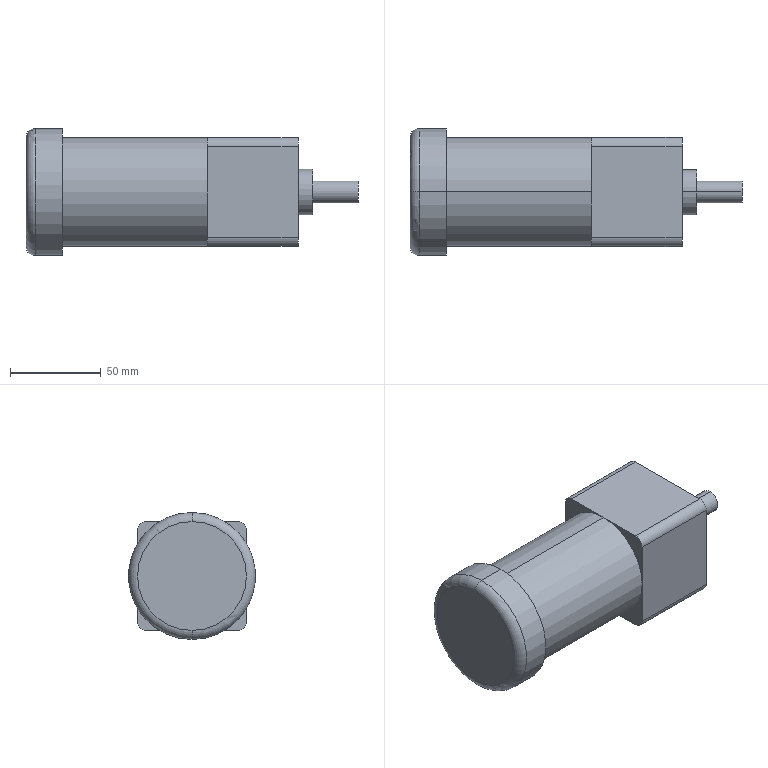Component | SolidWorks | Motor-1 | 1 solid | 27 faces | box 183 x 70 x 70 mm | volume 487703 mm3 | plane 13 | cylinder 12 | torus 2 | commonest cylinder face diameters 10 x4 12 x2 25 x2 70 x2 60 x2 | material Plain Carbon Steel
build123d program:
from build123d import *

# Parameters (mm, degrees)
SKETCH1_W           = 60
SKETCH1_H           = 60
BOSS_EXTRUDE1_DEPTH = 50
SKETCH2_R           = 30
BOSS_EXTRUDE2_DEPTH = 80
SKETCH3_R           = 35
BOSS_EXTRUDE3_DEPTH = 20
SKETCH4_R           = 12.5
BOSS_EXTRUDE4_DEPTH = 8
SKETCH5_R           = 6
BOSS_EXTRUDE5_DEPTH = 25
FILLET1_R           = 5


with BuildPart() as part:
    # Sketch1 → Boss-Extrude1 (new body)
    with BuildSketch(Plane.XY):
        Rectangle(SKETCH1_W, SKETCH1_H)
    extrude(amount=BOSS_EXTRUDE1_DEPTH)

    # Sketch2 → Boss-Extrude2 (add)
    with BuildSketch(Plane(origin=(0, 0, 0), x_dir=(-1, 0, 0), z_dir=(0, 0, -1))):
        Circle(SKETCH2_R)
    extrude(amount=BOSS_EXTRUDE2_DEPTH)

    # Sketch3 → Boss-Extrude3 (add)
    with BuildSketch(Plane(origin=(0, 0, -80), x_dir=(-1, 0, 0), z_dir=(0, 0, -1))):
        Circle(SKETCH3_R)
    extrude(amount=BOSS_EXTRUDE3_DEPTH)

    # Sketch4 → Boss-Extrude4 (add)
    with BuildSketch(Plane.XY.offset(50)):
        Circle(SKETCH4_R)
    extrude(amount=BOSS_EXTRUDE4_DEPTH)

    # Sketch5 → Boss-Extrude5 (add)
    with BuildSketch(Plane.XY.offset(58)):
        Circle(SKETCH5_R)
    extrude(amount=BOSS_EXTRUDE5_DEPTH)

    # Fillet1
    fillet1_edges = [part.edges().sort_by_distance(p)[0] for p in [
        (35, 0, -100),
        (-30, 30, 25),
        (30, 30, 25),
        (30, -30, 25),
        (-30, -30, 25),
    ]]
    fillet(fillet1_edges, radius=FILLET1_R)


solid = part.part

# Placed as in the assembly
solid = solid.moved(Location((-106.55, 5.646, 1535), (0, 90, 0)))
STEP:
#1=COLOUR_RGB('',0.7922,0.8196,0.9333);
#2=FILL_AREA_STYLE_COLOUR('',#1);
#3=FILL_AREA_STYLE('',(#2));
#4=SURFACE_STYLE_FILL_AREA(#3);
#5=SURFACE_SIDE_STYLE('',(#4));
#6=SURFACE_STYLE_USAGE(.BOTH.,#5);
#7=PRESENTATION_STYLE_ASSIGNMENT((#6));
#8=CARTESIAN_POINT('',(-7.935,0.2223,59.055));
#9=VERTEX_POINT('',#8);
#10=CARTESIAN_POINT('',(-7.935,0.2223,61.811));
#11=VERTEX_POINT('',#10);
#12=CARTESIAN_POINT('',(-7.935,0.2223,60.433));
#13=DIRECTION('',(1.,0.,0.));
#14=DIRECTION('',(0.,0.,1.));
#15=AXIS2_PLACEMENT_3D('',#12,#13,#14);
#16=CIRCLE('',#15,1.378);
#17=EDGE_CURVE('',#9,#11,#16,.T.);
#18=ORIENTED_EDGE('',*,*,#17,.F.);
#19=CARTESIAN_POINT('',(-8.132,0.2223,59.252));
#20=VERTEX_POINT('',#19);
#21=CARTESIAN_POINT('',(-7.935,0.2223,59.252));
#22=DIRECTION('',(-0.,1.,0.));
#23=DIRECTION('',(-1.,0.,0.));
#24=AXIS2_PLACEMENT_3D('',#21,#22,#23);
#25=CIRCLE('',#24,0.1969);
#26=EDGE_CURVE('',#9,#20,#25,.T.);
#27=ORIENTED_EDGE('',*,*,#26,.T.);
#28=CARTESIAN_POINT('',(-8.132,0.2223,61.614));
#29=VERTEX_POINT('',#28);
#30=CARTESIAN_POINT('',(-8.132,0.2223,60.433));
#31=DIRECTION('',(-1.,-0.,-0.));
#32=DIRECTION('',(0.,0.,1.));
#33=AXIS2_PLACEMENT_3D('',#30,#31,#32);
#34=CIRCLE('',#33,1.181);
#35=EDGE_CURVE('',#29,#20,#34,.T.);
#36=ORIENTED_EDGE('',*,*,#35,.F.);
#37=CARTESIAN_POINT('',(-7.935,0.2223,61.614));
#38=DIRECTION('',(0.,-1.,0.));
#39=DIRECTION('',(0.,-0.,-1.));
#40=AXIS2_PLACEMENT_3D('',#37,#38,#39);
#41=CIRCLE('',#40,0.1969);
#42=EDGE_CURVE('',#11,#29,#41,.T.);
#43=ORIENTED_EDGE('',*,*,#42,.F.);
#44=EDGE_LOOP('',(#18,#27,#36,#43));
#45=FACE_OUTER_BOUND('',#44,.T.);
#46=CARTESIAN_POINT('',(-7.935,0.2223,60.433));
#47=DIRECTION('',(-1.,-0.,-0.));
#48=DIRECTION('',(-0.,0.,1.));
#49=AXIS2_PLACEMENT_3D('',#46,#47,#48);
#50=TOROIDAL_SURFACE('',#49,1.181,0.1969);
#51=ADVANCED_FACE('',(#45),#50,.T.);
#52=CARTESIAN_POINT('',(-0.9271,0.2223,60.197));
#53=VERTEX_POINT('',#52);
#54=CARTESIAN_POINT('',(-0.9271,0.2223,60.669));
#55=VERTEX_POINT('',#54);
#56=CARTESIAN_POINT('',(-0.9271,0.2223,60.433));
#57=DIRECTION('',(1.,0.,0.));
#58=DIRECTION('',(0.,-0.,-1.));
#59=AXIS2_PLACEMENT_3D('',#56,#57,#58);
#60=CIRCLE('',#59,0.2362);
#61=EDGE_CURVE('',#53,#55,#60,.T.);
#62=ORIENTED_EDGE('',*,*,#61,.F.);
#63=CARTESIAN_POINT('',(-1.911,0.2223,60.197));
#64=VERTEX_POINT('',#63);
#65=CARTESIAN_POINT('',(-0.9271,0.2223,60.197));
#66=DIRECTION('',(-1.,-0.,-0.));
#67=VECTOR('',#66,39.37);
#68=LINE('',#65,#67);
#69=EDGE_CURVE('',#53,#64,#68,.T.);
#70=ORIENTED_EDGE('',*,*,#69,.T.);
#71=CARTESIAN_POINT('',(-1.911,0.2223,60.669));
#72=VERTEX_POINT('',#71);
#73=CARTESIAN_POINT('',(-1.911,0.2223,60.433));
#74=DIRECTION('',(1.,0.,0.));
#75=DIRECTION('',(0.,-0.,-1.));
#76=AXIS2_PLACEMENT_3D('',#73,#74,#75);
#77=CIRCLE('',#76,0.2362);
#78=EDGE_CURVE('',#64,#72,#77,.T.);
#79=ORIENTED_EDGE('',*,*,#78,.T.);
#80=CARTESIAN_POINT('',(-0.9271,0.2223,60.669));
#81=DIRECTION('',(-1.,-0.,-0.));
#82=VECTOR('',#81,39.37);
#83=LINE('',#80,#82);
#84=EDGE_CURVE('',#55,#72,#83,.T.);
#85=ORIENTED_EDGE('',*,*,#84,.F.);
#86=EDGE_LOOP('',(#62,#70,#79,#85));
#87=FACE_OUTER_BOUND('',#86,.T.);
#88=CARTESIAN_POINT('',(-0.9271,0.2223,60.433));
#89=DIRECTION('',(-1.,-0.,-0.));
#90=DIRECTION('',(0.,0.,1.));
#91=AXIS2_PLACEMENT_3D('',#88,#89,#90);
#92=CYLINDRICAL_SURFACE('',#91,0.2362);
#93=ADVANCED_FACE('',(#87),#92,.T.);
#94=CARTESIAN_POINT('',(-1.911,0.2223,59.941));
#95=VERTEX_POINT('',#94);
#96=CARTESIAN_POINT('',(-1.911,0.2223,60.925));
#97=VERTEX_POINT('',#96);
#98=CARTESIAN_POINT('',(-1.911,0.2223,60.433));
#99=DIRECTION('',(1.,0.,0.));
#100=DIRECTION('',(0.,-0.,-1.));
#101=AXIS2_PLACEMENT_3D('',#98,#99,#100);
#102=CIRCLE('',#101,0.4921);
#103=EDGE_CURVE('',#95,#97,#102,.T.);
#104=ORIENTED_EDGE('',*,*,#103,.F.);
#105=CARTESIAN_POINT('',(-2.226,0.2223,59.941));
#106=VERTEX_POINT('',#105);
#107=CARTESIAN_POINT('',(-1.911,0.2223,59.941));
#108=DIRECTION('',(-1.,-0.,-0.));
#109=VECTOR('',#108,39.37);
#110=LINE('',#107,#109);
#111=EDGE_CURVE('',#95,#106,#110,.T.);
#112=ORIENTED_EDGE('',*,*,#111,.T.);
#113=CARTESIAN_POINT('',(-2.226,0.2223,60.925));
#114=VERTEX_POINT('',#113);
#115=CARTESIAN_POINT('',(-2.226,0.2223,60.433));
#116=DIRECTION('',(1.,0.,0.));
#117=DIRECTION('',(0.,-0.,-1.));
#118=AXIS2_PLACEMENT_3D('',#115,#116,#117);
#119=CIRCLE('',#118,0.4921);
#120=EDGE_CURVE('',#106,#114,#119,.T.);
#121=ORIENTED_EDGE('',*,*,#120,.T.);
#122=CARTESIAN_POINT('',(-1.911,0.2223,60.925));
#123=DIRECTION('',(-1.,-0.,-0.));
#124=VECTOR('',#123,39.37);
#125=LINE('',#122,#124);
#126=EDGE_CURVE('',#97,#114,#125,.T.);
#127=ORIENTED_EDGE('',*,*,#126,.F.);
#128=EDGE_LOOP('',(#104,#112,#121,#127));
#129=FACE_OUTER_BOUND('',#128,.T.);
#130=CARTESIAN_POINT('',(-1.911,0.2223,60.433));
#131=DIRECTION('',(-1.,-0.,-0.));
#132=DIRECTION('',(0.,0.,1.));
#133=AXIS2_PLACEMENT_3D('',#130,#131,#132);
#134=CYLINDRICAL_SURFACE('',#133,0.4921);
#135=ADVANCED_FACE('',(#129),#134,.T.);
#136=ORIENTED_EDGE('',*,*,#17,.T.);
#137=CARTESIAN_POINT('',(-7.344,0.2223,61.811));
#138=VERTEX_POINT('',#137);
#139=CARTESIAN_POINT('',(-8.132,0.2223,61.811));
#140=DIRECTION('',(1.,0.,0.));
#141=VECTOR('',#140,39.37);
#142=LINE('',#139,#141);
#143=EDGE_CURVE('',#11,#138,#142,.T.);
#144=ORIENTED_EDGE('',*,*,#143,.T.);
#145=CARTESIAN_POINT('',(-7.344,0.2223,59.055));
#146=VERTEX_POINT('',#145);
#147=CARTESIAN_POINT('',(-7.344,0.2223,60.433));
#148=DIRECTION('',(-1.,-0.,-0.));
#149=DIRECTION('',(0.,0.,1.));
#150=AXIS2_PLACEMENT_3D('',#147,#148,#149);
#151=CIRCLE('',#150,1.378);
#152=EDGE_CURVE('',#138,#146,#151,.T.);
#153=ORIENTED_EDGE('',*,*,#152,.T.);
#154=CARTESIAN_POINT('',(-8.132,0.2223,59.055));
#155=DIRECTION('',(1.,0.,0.));
#156=VECTOR('',#155,39.37);
#157=LINE('',#154,#156);
#158=EDGE_CURVE('',#9,#146,#157,.T.);
#159=ORIENTED_EDGE('',*,*,#158,.F.);
#160=EDGE_LOOP('',(#136,#144,#153,#159));
#161=FACE_OUTER_BOUND('',#160,.T.);
#162=CARTESIAN_POINT('',(-8.132,0.2223,60.433));
#163=DIRECTION('',(1.,0.,0.));
#164=DIRECTION('',(0.,-0.,-1.));
#165=AXIS2_PLACEMENT_3D('',#162,#163,#164);
#166=CYLINDRICAL_SURFACE('',#165,1.378);
#167=ADVANCED_FACE('',(#161),#166,.T.);
#168=CARTESIAN_POINT('',(-7.344,0.2223,61.614));
#169=VERTEX_POINT('',#168);
#170=CARTESIAN_POINT('',(-7.344,0.2223,59.252));
#171=VERTEX_POINT('',#170);
#172=CARTESIAN_POINT('',(-7.344,0.2223,60.433));
#173=DIRECTION('',(-1.,-0.,-0.));
#174=DIRECTION('',(0.,0.,1.));
#175=AXIS2_PLACEMENT_3D('',#172,#173,#174);
#176=CIRCLE('',#175,1.181);
#177=EDGE_CURVE('',#169,#171,#176,.T.);
#178=ORIENTED_EDGE('',*,*,#177,.F.);
#179=CARTESIAN_POINT('',(-4.195,0.2223,61.614));
#180=VERTEX_POINT('',#179);
#181=CARTESIAN_POINT('',(-7.344,0.2223,61.614));
#182=DIRECTION('',(1.,0.,0.));
#183=VECTOR('',#182,39.37);
#184=LINE('',#181,#183);
#185=EDGE_CURVE('',#169,#180,#184,.T.);
#186=ORIENTED_EDGE('',*,*,#185,.T.);
#187=CARTESIAN_POINT('',(-4.195,1.403,60.433));
#188=VERTEX_POINT('',#187);
#189=CARTESIAN_POINT('',(-4.195,0.2223,60.433));
#190=DIRECTION('',(-1.,-0.,-0.));
#191=DIRECTION('',(0.,0.,1.));
#192=AXIS2_PLACEMENT_3D('',#189,#190,#191);
#193=CIRCLE('',#192,1.181);
#194=EDGE_CURVE('',#180,#188,#193,.T.);
#195=ORIENTED_EDGE('',*,*,#194,.T.);
#196=CARTESIAN_POINT('',(-4.195,0.2223,59.252));
#197=VERTEX_POINT('',#196);
#198=CARTESIAN_POINT('',(-4.195,0.2223,60.433));
#199=DIRECTION('',(-1.,-0.,-0.));
#200=DIRECTION('',(0.,0.,1.));
#201=AXIS2_PLACEMENT_3D('',#198,#199,#200);
#202=CIRCLE('',#201,1.181);
#203=EDGE_CURVE('',#188,#197,#202,.T.);
#204=ORIENTED_EDGE('',*,*,#203,.T.);
#205=CARTESIAN_POINT('',(-7.344,0.2223,59.252));
#206=DIRECTION('',(1.,0.,0.));
#207=VECTOR('',#206,39.37);
#208=LINE('',#205,#207);
#209=EDGE_CURVE('',#171,#197,#208,.T.);
#210=ORIENTED_EDGE('',*,*,#209,.F.);
#211=EDGE_LOOP('',(#178,#186,#195,#204,#210));
#212=FACE_OUTER_BOUND('',#211,.T.);
#213=CARTESIAN_POINT('',(-7.344,0.2223,60.433));
#214=DIRECTION('',(1.,0.,0.));
#215=DIRECTION('',(0.,-0.,-1.));
#216=AXIS2_PLACEMENT_3D('',#213,#214,#215);
#217=CYLINDRICAL_SURFACE('',#216,1.181);
#218=ADVANCED_FACE('',(#212),#217,.T.);
#219=CARTESIAN_POINT('',(-1.911,0.2223,60.433));
#220=DIRECTION('',(1.,0.,0.));
#221=DIRECTION('',(0.,-0.,-1.));
#222=AXIS2_PLACEMENT_3D('',#219,#220,#221);
#223=CIRCLE('',#222,0.4921);
#224=EDGE_CURVE('',#97,#95,#223,.T.);
#225=ORIENTED_EDGE('',*,*,#224,.T.);
#226=ORIENTED_EDGE('',*,*,#103,.T.);
#227=EDGE_LOOP('',(#225,#226));
#228=FACE_OUTER_BOUND('',#227,.T.);
#229=CARTESIAN_POINT('',(-1.911,0.2223,60.433));
#230=DIRECTION('',(1.,0.,0.));
#231=DIRECTION('',(0.,-0.,-1.));
#232=AXIS2_PLACEMENT_3D('',#229,#230,#231);
#233=CIRCLE('',#232,0.2362);
#234=EDGE_CURVE('',#72,#64,#233,.T.);
#235=ORIENTED_EDGE('',*,*,#234,.F.);
#236=ORIENTED_EDGE('',*,*,#78,.F.);
#237=EDGE_LOOP('',(#235,#236));
#238=FACE_BOUND('',#237,.T.);
#239=CARTESIAN_POINT('',(-1.911,0.2223,60.433));
#240=DIRECTION('',(1.,0.,0.));
#241=DIRECTION('',(0.,-0.,-1.));
#242=AXIS2_PLACEMENT_3D('',#239,#240,#241);
#243=PLANE('',#242);
#244=ADVANCED_FACE('',(#228,#238),#243,.T.);
#245=CARTESIAN_POINT('',(-2.226,-0.9588,61.417));
#246=VERTEX_POINT('',#245);
#247=CARTESIAN_POINT('',(-2.226,-0.9588,59.449));
#248=VERTEX_POINT('',#247);
#249=CARTESIAN_POINT('',(-2.226,-0.9588,59.252));
#250=DIRECTION('',(0.,-0.,-1.));
#251=VECTOR('',#250,39.37);
#252=LINE('',#249,#251);
#253=EDGE_CURVE('',#246,#248,#252,.T.);
#254=ORIENTED_EDGE('',*,*,#253,.T.);
#255=CARTESIAN_POINT('',(-2.226,-0.762,59.252));
#256=VERTEX_POINT('',#255);
#257=CARTESIAN_POINT('',(-2.226,-0.762,59.449));
#258=DIRECTION('',(1.,0.,0.));
#259=DIRECTION('',(0.,0.,-1.));
#260=AXIS2_PLACEMENT_3D('',#257,#258,#259);
#261=CIRCLE('',#260,0.1969);
#262=EDGE_CURVE('',#248,#256,#261,.T.);
#263=ORIENTED_EDGE('',*,*,#262,.T.);
#264=CARTESIAN_POINT('',(-2.226,1.207,59.252));
#265=VERTEX_POINT('',#264);
#266=CARTESIAN_POINT('',(-2.226,-0.9588,59.252));
#267=DIRECTION('',(-0.,1.,-0.));
#268=VECTOR('',#267,39.37);
#269=LINE('',#266,#268);
#270=EDGE_CURVE('',#256,#265,#269,.T.);
#271=ORIENTED_EDGE('',*,*,#270,.T.);
#272=CARTESIAN_POINT('',(-2.226,1.403,59.449));
#273=VERTEX_POINT('',#272);
#274=CARTESIAN_POINT('',(-2.226,1.207,59.449));
#275=DIRECTION('',(1.,0.,0.));
#276=DIRECTION('',(0.,0.,-1.));
#277=AXIS2_PLACEMENT_3D('',#274,#275,#276);
#278=CIRCLE('',#277,0.1969);
#279=EDGE_CURVE('',#265,#273,#278,.T.);
#280=ORIENTED_EDGE('',*,*,#279,.T.);
#281=CARTESIAN_POINT('',(-2.226,1.403,61.417));
#282=VERTEX_POINT('',#281);
#283=CARTESIAN_POINT('',(-2.226,1.403,59.252));
#284=DIRECTION('',(-0.,0.,1.));
#285=VECTOR('',#284,39.37);
#286=LINE('',#283,#285);
#287=EDGE_CURVE('',#273,#282,#286,.T.);
#288=ORIENTED_EDGE('',*,*,#287,.T.);
#289=CARTESIAN_POINT('',(-2.226,1.207,61.614));
#290=VERTEX_POINT('',#289);
#291=CARTESIAN_POINT('',(-2.226,1.207,61.417));
#292=DIRECTION('',(1.,0.,0.));
#293=DIRECTION('',(0.,0.,-1.));
#294=AXIS2_PLACEMENT_3D('',#291,#292,#293);
#295=CIRCLE('',#294,0.1969);
#296=EDGE_CURVE('',#282,#290,#295,.T.);
#297=ORIENTED_EDGE('',*,*,#296,.T.);
#298=CARTESIAN_POINT('',(-2.226,-0.762,61.614));
#299=VERTEX_POINT('',#298);
#300=CARTESIAN_POINT('',(-2.226,-0.9588,61.614));
#301=DIRECTION('',(0.,-1.,0.));
#302=VECTOR('',#301,39.37);
#303=LINE('',#300,#302);
#304=EDGE_CURVE('',#290,#299,#303,.T.);
#305=ORIENTED_EDGE('',*,*,#304,.T.);
#306=CARTESIAN_POINT('',(-2.226,-0.762,61.417));
#307=DIRECTION('',(1.,0.,0.));
#308=DIRECTION('',(0.,0.,-1.));
#309=AXIS2_PLACEMENT_3D('',#306,#307,#308);
#310=CIRCLE('',#309,0.1969);
#311=EDGE_CURVE('',#299,#246,#310,.T.);
#312=ORIENTED_EDGE('',*,*,#311,.T.);
#313=EDGE_LOOP('',(#254,#263,#271,#280,#288,#297,#305,#312));
#314=FACE_OUTER_BOUND('',#313,.T.);
#315=CARTESIAN_POINT('',(-2.226,0.2223,60.433));
#316=DIRECTION('',(1.,0.,0.));
#317=DIRECTION('',(0.,-0.,-1.));
#318=AXIS2_PLACEMENT_3D('',#315,#316,#317);
#319=CIRCLE('',#318,0.4921);
#320=EDGE_CURVE('',#114,#106,#319,.T.);
#321=ORIENTED_EDGE('',*,*,#320,.F.);
#322=ORIENTED_EDGE('',*,*,#120,.F.);
#323=EDGE_LOOP('',(#321,#322));
#324=FACE_BOUND('',#323,.T.);
#325=CARTESIAN_POINT('',(-2.226,0.2223,60.433));
#326=DIRECTION('',(1.,0.,0.));
#327=DIRECTION('',(0.,-0.,-1.));
#328=AXIS2_PLACEMENT_3D('',#325,#326,#327);
#329=PLANE('',#328);
#330=ADVANCED_FACE('',(#314,#324),#329,.T.);
#331=CARTESIAN_POINT('',(-4.195,1.207,61.614));
#332=VERTEX_POINT('',#331);
#333=CARTESIAN_POINT('',(-4.195,-0.9588,61.614));
#334=DIRECTION('',(0.,-1.,0.));
#335=VECTOR('',#334,39.37);
#336=LINE('',#333,#335);
#337=EDGE_CURVE('',#332,#180,#336,.T.);
#338=ORIENTED_EDGE('',*,*,#337,.F.);
#339=CARTESIAN_POINT('',(-4.195,1.403,61.417));
#340=VERTEX_POINT('',#339);
#341=CARTESIAN_POINT('',(-4.195,1.207,61.417));
#342=DIRECTION('',(-1.,-0.,-0.));
#343=DIRECTION('',(0.,0.,-1.));
#344=AXIS2_PLACEMENT_3D('',#341,#342,#343);
#345=CIRCLE('',#344,0.1969);
#346=EDGE_CURVE('',#332,#340,#345,.T.);
#347=ORIENTED_EDGE('',*,*,#346,.T.);
#348=CARTESIAN_POINT('',(-4.195,1.403,59.252));
#349=DIRECTION('',(-0.,0.,1.));
#350=VECTOR('',#349,39.37);
#351=LINE('',#348,#350);
#352=EDGE_CURVE('',#188,#340,#351,.T.);
#353=ORIENTED_EDGE('',*,*,#352,.F.);
#354=ORIENTED_EDGE('',*,*,#194,.F.);
#355=EDGE_LOOP('',(#338,#347,#353,#354));
#356=FACE_OUTER_BOUND('',#355,.T.);
#357=CARTESIAN_POINT('',(-4.195,0.2223,60.433));
#358=DIRECTION('',(1.,0.,0.));
#359=DIRECTION('',(0.,-0.,-1.));
#360=AXIS2_PLACEMENT_3D('',#357,#358,#359);
#361=PLANE('',#360);
#362=ADVANCED_FACE('',(#356),#361,.F.);
#363=CARTESIAN_POINT('',(-4.195,1.403,59.449));
#364=VERTEX_POINT('',#363);
#365=CARTESIAN_POINT('',(-4.195,1.403,59.252));
#366=DIRECTION('',(-0.,0.,1.));
#367=VECTOR('',#366,39.37);
#368=LINE('',#365,#367);
#369=EDGE_CURVE('',#364,#188,#368,.T.);
#370=ORIENTED_EDGE('',*,*,#369,.F.);
#371=CARTESIAN_POINT('',(-4.195,1.207,59.252));
#372=VERTEX_POINT('',#371);
#373=CARTESIAN_POINT('',(-4.195,1.207,59.449));
#374=DIRECTION('',(-1.,-0.,-0.));
#375=DIRECTION('',(0.,0.,-1.));
#376=AXIS2_PLACEMENT_3D('',#373,#374,#375);
#377=CIRCLE('',#376,0.1969);
#378=EDGE_CURVE('',#364,#372,#377,.T.);
#379=ORIENTED_EDGE('',*,*,#378,.T.);
#380=CARTESIAN_POINT('',(-4.195,-0.9588,59.252));
#381=DIRECTION('',(-0.,1.,-0.));
#382=VECTOR('',#381,39.37);
#383=LINE('',#380,#382);
#384=EDGE_CURVE('',#197,#372,#383,.T.);
#385=ORIENTED_EDGE('',*,*,#384,.F.);
#386=ORIENTED_EDGE('',*,*,#203,.F.);
#387=EDGE_LOOP('',(#370,#379,#385,#386));
#388=FACE_OUTER_BOUND('',#387,.T.);
#389=CARTESIAN_POINT('',(-4.195,0.2223,60.433));
#390=DIRECTION('',(1.,0.,0.));
#391=DIRECTION('',(0.,-0.,-1.));
#392=AXIS2_PLACEMENT_3D('',#389,#390,#391);
#393=PLANE('',#392);
#394=ADVANCED_FACE('',(#388),#393,.F.);
#395=CARTESIAN_POINT('',(-4.195,-0.762,59.252));
#396=VERTEX_POINT('',#395);
#397=CARTESIAN_POINT('',(-4.195,-0.9588,59.252));
#398=DIRECTION('',(-0.,1.,-0.));
#399=VECTOR('',#398,39.37);
#400=LINE('',#397,#399);
#401=EDGE_CURVE('',#396,#197,#400,.T.);
#402=ORIENTED_EDGE('',*,*,#401,.F.);
#403=CARTESIAN_POINT('',(-4.195,-0.9588,59.449));
#404=VERTEX_POINT('',#403);
#405=CARTESIAN_POINT('',(-4.195,-0.762,59.449));
#406=DIRECTION('',(-1.,-0.,-0.));
#407=DIRECTION('',(0.,0.,-1.));
#408=AXIS2_PLACEMENT_3D('',#405,#406,#407);
#409=CIRCLE('',#408,0.1969);
#410=EDGE_CURVE('',#396,#404,#409,.T.);
#411=ORIENTED_EDGE('',*,*,#410,.T.);
#412=CARTESIAN_POINT('',(-4.195,-0.9588,60.433));
#413=VERTEX_POINT('',#412);
#414=CARTESIAN_POINT('',(-4.195,-0.9588,59.252));
#415=DIRECTION('',(0.,-0.,-1.));
#416=VECTOR('',#415,39.37);
#417=LINE('',#414,#416);
#418=EDGE_CURVE('',#413,#404,#417,.T.);
#419=ORIENTED_EDGE('',*,*,#418,.F.);
#420=CARTESIAN_POINT('',(-4.195,0.2223,60.433));
#421=DIRECTION('',(-1.,-0.,-0.));
#422=DIRECTION('',(0.,0.,1.));
#423=AXIS2_PLACEMENT_3D('',#420,#421,#422);
#424=CIRCLE('',#423,1.181);
#425=EDGE_CURVE('',#197,#413,#424,.T.);
#426=ORIENTED_EDGE('',*,*,#425,.F.);
#427=EDGE_LOOP('',(#402,#411,#419,#426));
#428=FACE_OUTER_BOUND('',#427,.T.);
#429=CARTESIAN_POINT('',(-4.195,0.2223,60.433));
#430=DIRECTION('',(1.,0.,0.));
#431=DIRECTION('',(0.,-0.,-1.));
#432=AXIS2_PLACEMENT_3D('',#429,#430,#431);
#433=PLANE('',#432);
#434=ADVANCED_FACE('',(#428),#433,.F.);
#435=CARTESIAN_POINT('',(-4.195,-0.9588,61.417));
#436=VERTEX_POINT('',#435);
#437=CARTESIAN_POINT('',(-4.195,-0.9588,59.252));
#438=DIRECTION('',(0.,-0.,-1.));
#439=VECTOR('',#438,39.37);
#440=LINE('',#437,#439);
#441=EDGE_CURVE('',#436,#413,#440,.T.);
#442=ORIENTED_EDGE('',*,*,#441,.F.);
#443=CARTESIAN_POINT('',(-4.195,-0.762,61.614));
#444=VERTEX_POINT('',#443);
#445=CARTESIAN_POINT('',(-4.195,-0.762,61.417));
#446=DIRECTION('',(-1.,-0.,-0.));
#447=DIRECTION('',(0.,0.,-1.));
#448=AXIS2_PLACEMENT_3D('',#445,#446,#447);
#449=CIRCLE('',#448,0.1969);
#450=EDGE_CURVE('',#436,#444,#449,.T.);
#451=ORIENTED_EDGE('',*,*,#450,.T.);
#452=CARTESIAN_POINT('',(-4.195,-0.9588,61.614));
#453=DIRECTION('',(0.,-1.,0.));
#454=VECTOR('',#453,39.37);
#455=LINE('',#452,#454);
#456=EDGE_CURVE('',#180,#444,#455,.T.);
#457=ORIENTED_EDGE('',*,*,#456,.F.);
#458=CARTESIAN_POINT('',(-4.195,0.2223,60.433));
#459=DIRECTION('',(-1.,-0.,-0.));
#460=DIRECTION('',(0.,0.,1.));
#461=AXIS2_PLACEMENT_3D('',#458,#459,#460);
#462=CIRCLE('',#461,1.181);
#463=EDGE_CURVE('',#413,#180,#462,.T.);
#464=ORIENTED_EDGE('',*,*,#463,.F.);
#465=EDGE_LOOP('',(#442,#451,#457,#464));
#466=FACE_OUTER_BOUND('',#465,.T.);
#467=CARTESIAN_POINT('',(-4.195,0.2223,60.433));
#468=DIRECTION('',(1.,0.,0.));
#469=DIRECTION('',(0.,-0.,-1.));
#470=AXIS2_PLACEMENT_3D('',#467,#468,#469);
#471=PLANE('',#470);
#472=ADVANCED_FACE('',(#466),#471,.F.);
#473=ORIENTED_EDGE('',*,*,#456,.T.);
#474=CARTESIAN_POINT('',(-2.226,-0.762,61.614));
#475=DIRECTION('',(1.,0.,0.));
#476=VECTOR('',#475,39.37);
#477=LINE('',#474,#476);
#478=EDGE_CURVE('',#444,#299,#477,.T.);
#479=ORIENTED_EDGE('',*,*,#478,.T.);
#480=ORIENTED_EDGE('',*,*,#304,.F.);
#481=CARTESIAN_POINT('',(-2.226,1.207,61.614));
#482=DIRECTION('',(-1.,-0.,-0.));
#483=VECTOR('',#482,39.37);
#484=LINE('',#481,#483);
#485=EDGE_CURVE('',#290,#332,#484,.T.);
#486=ORIENTED_EDGE('',*,*,#485,.T.);
#487=ORIENTED_EDGE('',*,*,#337,.T.);
#488=EDGE_LOOP('',(#473,#479,#480,#486,#487));
#489=FACE_OUTER_BOUND('',#488,.T.);
#490=CARTESIAN_POINT('',(-2.226,-0.9588,61.614));
#491=DIRECTION('',(0.,-0.,-1.));
#492=DIRECTION('',(-1.,-0.,-0.));
#493=AXIS2_PLACEMENT_3D('',#490,#491,#492);
#494=PLANE('',#493);
#495=ADVANCED_FACE('',(#489),#494,.F.);
#496=ORIENTED_EDGE('',*,*,#418,.T.);
#497=CARTESIAN_POINT('',(-2.226,-0.9588,59.449));
#498=DIRECTION('',(1.,0.,0.));
#499=VECTOR('',#498,39.37);
#500=LINE('',#497,#499);
#501=EDGE_CURVE('',#404,#248,#500,.T.);
#502=ORIENTED_EDGE('',*,*,#501,.T.);
#503=ORIENTED_EDGE('',*,*,#253,.F.);
#504=CARTESIAN_POINT('',(-2.226,-0.9588,61.417));
#505=DIRECTION('',(-1.,-0.,-0.));
#506=VECTOR('',#505,39.37);
#507=LINE('',#504,#506);
#508=EDGE_CURVE('',#246,#436,#507,.T.);
#509=ORIENTED_EDGE('',*,*,#508,.T.);
#510=ORIENTED_EDGE('',*,*,#441,.T.);
#511=EDGE_LOOP('',(#496,#502,#503,#509,#510));
#512=FACE_OUTER_BOUND('',#511,.T.);
#513=CARTESIAN_POINT('',(-2.226,-0.9588,59.252));
#514=DIRECTION('',(-0.,1.,-0.));
#515=DIRECTION('',(1.,0.,0.));
#516=AXIS2_PLACEMENT_3D('',#513,#514,#515);
#517=PLANE('',#516);
#518=ADVANCED_FACE('',(#512),#517,.F.);
#519=ORIENTED_EDGE('',*,*,#270,.F.);
#520=CARTESIAN_POINT('',(-2.226,-0.762,59.252));
#521=DIRECTION('',(-1.,-0.,-0.));
#522=VECTOR('',#521,39.37);
#523=LINE('',#520,#522);
#524=EDGE_CURVE('',#256,#396,#523,.T.);
#525=ORIENTED_EDGE('',*,*,#524,.T.);
#526=ORIENTED_EDGE('',*,*,#401,.T.);
#527=ORIENTED_EDGE('',*,*,#384,.T.);
#528=CARTESIAN_POINT('',(-2.226,1.207,59.252));
#529=DIRECTION('',(1.,0.,0.));
#530=VECTOR('',#529,39.37);
#531=LINE('',#528,#530);
#532=EDGE_CURVE('',#372,#265,#531,.T.);
#533=ORIENTED_EDGE('',*,*,#532,.T.);
#534=EDGE_LOOP('',(#519,#525,#526,#527,#533));
#535=FACE_OUTER_BOUND('',#534,.T.);
#536=CARTESIAN_POINT('',(-2.226,-0.9588,59.252));
#537=DIRECTION('',(-0.,0.,1.));
#538=DIRECTION('',(1.,0.,0.));
#539=AXIS2_PLACEMENT_3D('',#536,#537,#538);
#540=PLANE('',#539);
#541=ADVANCED_FACE('',(#535),#540,.F.);
#542=ORIENTED_EDGE('',*,*,#352,.T.);
#543=CARTESIAN_POINT('',(-2.226,1.403,61.417));
#544=DIRECTION('',(1.,0.,0.));
#545=VECTOR('',#544,39.37);
#546=LINE('',#543,#545);
#547=EDGE_CURVE('',#340,#282,#546,.T.);
#548=ORIENTED_EDGE('',*,*,#547,.T.);
#549=ORIENTED_EDGE('',*,*,#287,.F.);
#550=CARTESIAN_POINT('',(-2.226,1.403,59.449));
#551=DIRECTION('',(-1.,-0.,-0.));
#552=VECTOR('',#551,39.37);
#553=LINE('',#550,#552);
#554=EDGE_CURVE('',#273,#364,#553,.T.);
#555=ORIENTED_EDGE('',*,*,#554,.T.);
#556=ORIENTED_EDGE('',*,*,#369,.T.);
#557=EDGE_LOOP('',(#542,#548,#549,#555,#556));
#558=FACE_OUTER_BOUND('',#557,.T.);
#559=CARTESIAN_POINT('',(-2.226,1.403,59.252));
#560=DIRECTION('',(0.,-1.,0.));
#561=DIRECTION('',(-1.,-0.,-0.));
#562=AXIS2_PLACEMENT_3D('',#559,#560,#561);
#563=PLANE('',#562);
#564=ADVANCED_FACE('',(#558),#563,.F.);
#565=ORIENTED_EDGE('',*,*,#185,.F.);
#566=CARTESIAN_POINT('',(-7.344,0.2223,60.433));
#567=DIRECTION('',(-1.,-0.,-0.));
#568=DIRECTION('',(0.,0.,1.));
#569=AXIS2_PLACEMENT_3D('',#566,#567,#568);
#570=CIRCLE('',#569,1.181);
#571=EDGE_CURVE('',#171,#169,#570,.T.);
#572=ORIENTED_EDGE('',*,*,#571,.F.);
#573=ORIENTED_EDGE('',*,*,#209,.T.);
#574=ORIENTED_EDGE('',*,*,#425,.T.);
#575=ORIENTED_EDGE('',*,*,#463,.T.);
#576=EDGE_LOOP('',(#565,#572,#573,#574,#575));
#577=FACE_OUTER_BOUND('',#576,.T.);
#578=CARTESIAN_POINT('',(-7.344,0.2223,60.433));
#579=DIRECTION('',(1.,0.,0.));
#580=DIRECTION('',(0.,-0.,-1.));
#581=AXIS2_PLACEMENT_3D('',#578,#579,#580);
#582=CYLINDRICAL_SURFACE('',#581,1.181);
#583=ADVANCED_FACE('',(#577),#582,.T.);
#584=CARTESIAN_POINT('',(-7.344,0.2223,60.433));
#585=DIRECTION('',(-1.,-0.,-0.));
#586=DIRECTION('',(0.,0.,1.));
#587=AXIS2_PLACEMENT_3D('',#584,#585,#586);
#588=CIRCLE('',#587,1.378);
#589=EDGE_CURVE('',#146,#138,#588,.T.);
#590=ORIENTED_EDGE('',*,*,#589,.F.);
#591=ORIENTED_EDGE('',*,*,#152,.F.);
#592=EDGE_LOOP('',(#590,#591));
#593=FACE_OUTER_BOUND('',#592,.T.);
#594=ORIENTED_EDGE('',*,*,#571,.T.);
#595=ORIENTED_EDGE('',*,*,#177,.T.);
#596=EDGE_LOOP('',(#594,#595));
#597=FACE_BOUND('',#596,.T.);
#598=CARTESIAN_POINT('',(-7.344,0.2223,60.433));
#599=DIRECTION('',(-1.,-0.,-0.));
#600=DIRECTION('',(-0.,0.,1.));
#601=AXIS2_PLACEMENT_3D('',#598,#599,#600);
#602=PLANE('',#601);
#603=ADVANCED_FACE('',(#593,#597),#602,.F.);
#604=ORIENTED_EDGE('',*,*,#143,.F.);
#605=CARTESIAN_POINT('',(-7.935,0.2223,60.433));
#606=DIRECTION('',(1.,0.,0.));
#607=DIRECTION('',(0.,0.,1.));
#608=AXIS2_PLACEMENT_3D('',#605,#606,#607);
#609=CIRCLE('',#608,1.378);
#610=EDGE_CURVE('',#11,#9,#609,.T.);
#611=ORIENTED_EDGE('',*,*,#610,.T.);
#612=ORIENTED_EDGE('',*,*,#158,.T.);
#613=ORIENTED_EDGE('',*,*,#589,.T.);
#614=EDGE_LOOP('',(#604,#611,#612,#613));
#615=FACE_OUTER_BOUND('',#614,.T.);
#616=CARTESIAN_POINT('',(-8.132,0.2223,60.433));
#617=DIRECTION('',(1.,0.,0.));
#618=DIRECTION('',(0.,-0.,-1.));
#619=AXIS2_PLACEMENT_3D('',#616,#617,#618);
#620=CYLINDRICAL_SURFACE('',#619,1.378);
#621=ADVANCED_FACE('',(#615),#620,.T.);
#622=ORIENTED_EDGE('',*,*,#35,.T.);
#623=CARTESIAN_POINT('',(-8.132,0.2223,60.433));
#624=DIRECTION('',(-1.,-0.,-0.));
#625=DIRECTION('',(0.,0.,1.));
#626=AXIS2_PLACEMENT_3D('',#623,#624,#625);
#627=CIRCLE('',#626,1.181);
#628=EDGE_CURVE('',#20,#29,#627,.T.);
#629=ORIENTED_EDGE('',*,*,#628,.T.);
#630=EDGE_LOOP('',(#622,#629));
#631=FACE_OUTER_BOUND('',#630,.T.);
#632=CARTESIAN_POINT('',(-8.132,0.2223,60.433));
#633=DIRECTION('',(-1.,-0.,-0.));
#634=DIRECTION('',(-0.,0.,1.));
#635=AXIS2_PLACEMENT_3D('',#632,#633,#634);
#636=PLANE('',#635);
#637=ADVANCED_FACE('',(#631),#636,.T.);
#638=ORIENTED_EDGE('',*,*,#111,.F.);
#639=ORIENTED_EDGE('',*,*,#224,.F.);
#640=ORIENTED_EDGE('',*,*,#126,.T.);
#641=ORIENTED_EDGE('',*,*,#320,.T.);
#642=EDGE_LOOP('',(#638,#639,#640,#641));
#643=FACE_OUTER_BOUND('',#642,.T.);
#644=CARTESIAN_POINT('',(-1.911,0.2223,60.433));
#645=DIRECTION('',(-1.,-0.,-0.));
#646=DIRECTION('',(0.,0.,1.));
#647=AXIS2_PLACEMENT_3D('',#644,#645,#646);
#648=CYLINDRICAL_SURFACE('',#647,0.4921);
#649=ADVANCED_FACE('',(#643),#648,.T.);
#650=ORIENTED_EDGE('',*,*,#69,.F.);
#651=CARTESIAN_POINT('',(-0.9271,0.2223,60.433));
#652=DIRECTION('',(1.,0.,0.));
#653=DIRECTION('',(0.,-0.,-1.));
#654=AXIS2_PLACEMENT_3D('',#651,#652,#653);
#655=CIRCLE('',#654,0.2362);
#656=EDGE_CURVE('',#55,#53,#655,.T.);
#657=ORIENTED_EDGE('',*,*,#656,.F.);
#658=ORIENTED_EDGE('',*,*,#84,.T.);
#659=ORIENTED_EDGE('',*,*,#234,.T.);
#660=EDGE_LOOP('',(#650,#657,#658,#659));
#661=FACE_OUTER_BOUND('',#660,.T.);
#662=CARTESIAN_POINT('',(-0.9271,0.2223,60.433));
#663=DIRECTION('',(-1.,-0.,-0.));
#664=DIRECTION('',(0.,0.,1.));
#665=AXIS2_PLACEMENT_3D('',#662,#663,#664);
#666=CYLINDRICAL_SURFACE('',#665,0.2362);
#667=ADVANCED_FACE('',(#661),#666,.T.);
#668=ORIENTED_EDGE('',*,*,#656,.T.);
#669=ORIENTED_EDGE('',*,*,#61,.T.);
#670=EDGE_LOOP('',(#668,#669));
#671=FACE_OUTER_BOUND('',#670,.T.);
#672=CARTESIAN_POINT('',(-0.9271,0.2223,60.433));
#673=DIRECTION('',(1.,0.,0.));
#674=DIRECTION('',(0.,-0.,-1.));
#675=AXIS2_PLACEMENT_3D('',#672,#673,#674);
#676=PLANE('',#675);
#677=ADVANCED_FACE('',(#671),#676,.T.);
#678=ORIENTED_EDGE('',*,*,#26,.F.);
#679=ORIENTED_EDGE('',*,*,#610,.F.);
#680=ORIENTED_EDGE('',*,*,#42,.T.);
#681=ORIENTED_EDGE('',*,*,#628,.F.);
#682=EDGE_LOOP('',(#678,#679,#680,#681));
#683=FACE_OUTER_BOUND('',#682,.T.);
#684=CARTESIAN_POINT('',(-7.935,0.2223,60.433));
#685=DIRECTION('',(-1.,-0.,-0.));
#686=DIRECTION('',(-0.,0.,1.));
#687=AXIS2_PLACEMENT_3D('',#684,#685,#686);
#688=TOROIDAL_SURFACE('',#687,1.181,0.1969);
#689=ADVANCED_FACE('',(#683),#688,.T.);
#690=ORIENTED_EDGE('',*,*,#262,.F.);
#691=ORIENTED_EDGE('',*,*,#501,.F.);
#692=ORIENTED_EDGE('',*,*,#410,.F.);
#693=ORIENTED_EDGE('',*,*,#524,.F.);
#694=EDGE_LOOP('',(#690,#691,#692,#693));
#695=FACE_OUTER_BOUND('',#694,.T.);
#696=CARTESIAN_POINT('',(-2.226,-0.762,59.449));
#697=DIRECTION('',(-1.,-0.,-0.));
#698=DIRECTION('',(0.,0.,1.));
#699=AXIS2_PLACEMENT_3D('',#696,#697,#698);
#700=CYLINDRICAL_SURFACE('',#699,0.1969);
#701=ADVANCED_FACE('',(#695),#700,.T.);
#702=ORIENTED_EDGE('',*,*,#311,.F.);
#703=ORIENTED_EDGE('',*,*,#478,.F.);
#704=ORIENTED_EDGE('',*,*,#450,.F.);
#705=ORIENTED_EDGE('',*,*,#508,.F.);
#706=EDGE_LOOP('',(#702,#703,#704,#705));
#707=FACE_OUTER_BOUND('',#706,.T.);
#708=CARTESIAN_POINT('',(-2.226,-0.762,61.417));
#709=DIRECTION('',(-1.,-0.,-0.));
#710=DIRECTION('',(0.,0.,1.));
#711=AXIS2_PLACEMENT_3D('',#708,#709,#710);
#712=CYLINDRICAL_SURFACE('',#711,0.1969);
#713=ADVANCED_FACE('',(#707),#712,.T.);
#714=ORIENTED_EDGE('',*,*,#296,.F.);
#715=ORIENTED_EDGE('',*,*,#547,.F.);
#716=ORIENTED_EDGE('',*,*,#346,.F.);
#717=ORIENTED_EDGE('',*,*,#485,.F.);
#718=EDGE_LOOP('',(#714,#715,#716,#717));
#719=FACE_OUTER_BOUND('',#718,.T.);
#720=CARTESIAN_POINT('',(-2.226,1.207,61.417));
#721=DIRECTION('',(-1.,-0.,-0.));
#722=DIRECTION('',(0.,0.,1.));
#723=AXIS2_PLACEMENT_3D('',#720,#721,#722);
#724=CYLINDRICAL_SURFACE('',#723,0.1969);
#725=ADVANCED_FACE('',(#719),#724,.T.);
#726=ORIENTED_EDGE('',*,*,#279,.F.);
#727=ORIENTED_EDGE('',*,*,#532,.F.);
#728=ORIENTED_EDGE('',*,*,#378,.F.);
#729=ORIENTED_EDGE('',*,*,#554,.F.);
#730=EDGE_LOOP('',(#726,#727,#728,#729));
#731=FACE_OUTER_BOUND('',#730,.T.);
#732=CARTESIAN_POINT('',(-2.226,1.207,59.449));
#733=DIRECTION('',(-1.,-0.,-0.));
#734=DIRECTION('',(0.,0.,1.));
#735=AXIS2_PLACEMENT_3D('',#732,#733,#734);
#736=CYLINDRICAL_SURFACE('',#735,0.1969);
#737=ADVANCED_FACE('',(#731),#736,.T.);
#738=CLOSED_SHELL('',(#51,#93,#135,#167,#218,#244,#330,#362,#394,#434,#472,#495,#518,#541,#564,#583,#603,#621,#637,#649,#667,#677,#689,#701,#713,#725,#737));
#739=MANIFOLD_SOLID_BREP('',#738);
#740=STYLED_ITEM('',(#7),#739);
#741=(LENGTH_UNIT()NAMED_UNIT(*)SI_UNIT($,.METRE.));
#742=LENGTH_MEASURE_WITH_UNIT(LENGTH_MEASURE(0.0254),#741);
#743=DIMENSIONAL_EXPONENTS(1.,0.,0.,0.,0.,0.,0.);
#744=(CONVERSION_BASED_UNIT('',#742)LENGTH_UNIT()NAMED_UNIT(#743));
#745=UNCERTAINTY_MEASURE_WITH_UNIT(LENGTH_MEASURE(0.00001),#744,'','');
#746=(NAMED_UNIT(*)PLANE_ANGLE_UNIT()SI_UNIT($,.RADIAN.));
#747=(NAMED_UNIT(*)SI_UNIT($,.STERADIAN.)SOLID_ANGLE_UNIT());
#748=(GEOMETRIC_REPRESENTATION_CONTEXT(3)GLOBAL_UNCERTAINTY_ASSIGNED_CONTEXT((#745))GLOBAL_UNIT_ASSIGNED_CONTEXT((#744,#746,#747))REPRESENTATION_CONTEXT('',''));
#749=MECHANICAL_DESIGN_GEOMETRIC_PRESENTATION_REPRESENTATION('',(#740),#748);
#750=CARTESIAN_POINT('',(0.,0.,0.));
#751=DIRECTION('',(0.,0.,1.));
#752=DIRECTION('',(1.,0.,0.));
#753=AXIS2_PLACEMENT_3D('',#750,#751,#752);
#754=(LENGTH_UNIT()NAMED_UNIT(*)SI_UNIT($,.METRE.));
#755=LENGTH_MEASURE_WITH_UNIT(LENGTH_MEASURE(0.0254),#754);
#756=DIMENSIONAL_EXPONENTS(1.,0.,0.,0.,0.,0.,0.);
#757=(CONVERSION_BASED_UNIT('',#755)LENGTH_UNIT()NAMED_UNIT(#756));
#758=UNCERTAINTY_MEASURE_WITH_UNIT(LENGTH_MEASURE(0.00001),#757,'','');
#759=(NAMED_UNIT(*)PLANE_ANGLE_UNIT()SI_UNIT($,.RADIAN.));
#760=(NAMED_UNIT(*)SI_UNIT($,.STERADIAN.)SOLID_ANGLE_UNIT());
#761=(GEOMETRIC_REPRESENTATION_CONTEXT(3)GLOBAL_UNCERTAINTY_ASSIGNED_CONTEXT((#758))GLOBAL_UNIT_ASSIGNED_CONTEXT((#757,#759,#760))REPRESENTATION_CONTEXT('',''));
#762=ADVANCED_BREP_SHAPE_REPRESENTATION('',(#739,#753),#761);
#763=PRESENTATION_LAYER_ASSIGNMENT('','',(#740));